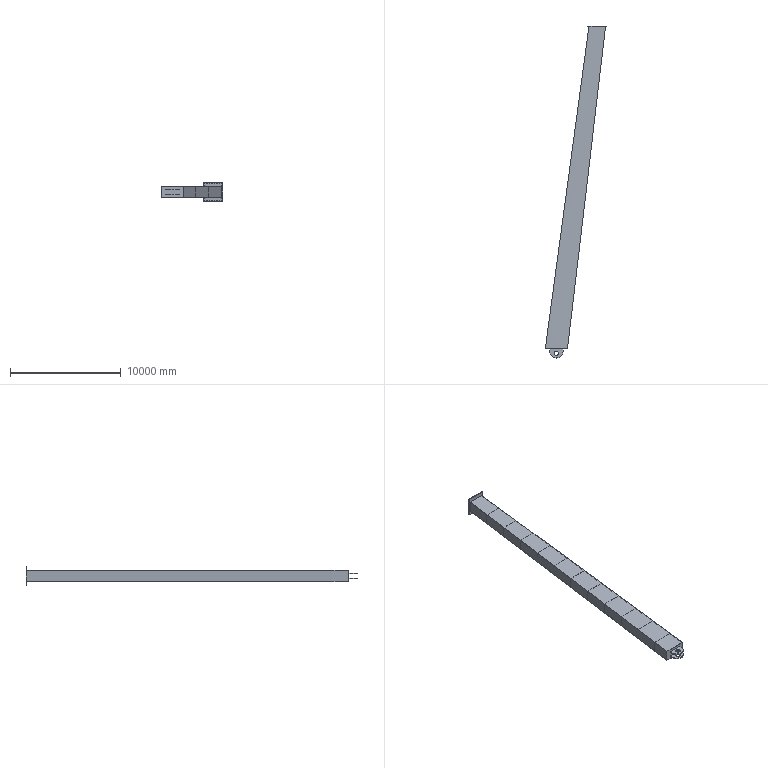Component | SolidWorks | FlexibleLegGenuine-3 | 1 solid | 181 faces | volume 7566859951 mm3 | plane 93 | cylinder 64 | spline 24 | commonest cylinder face diameters 40 x56 400 x4 1200 x4